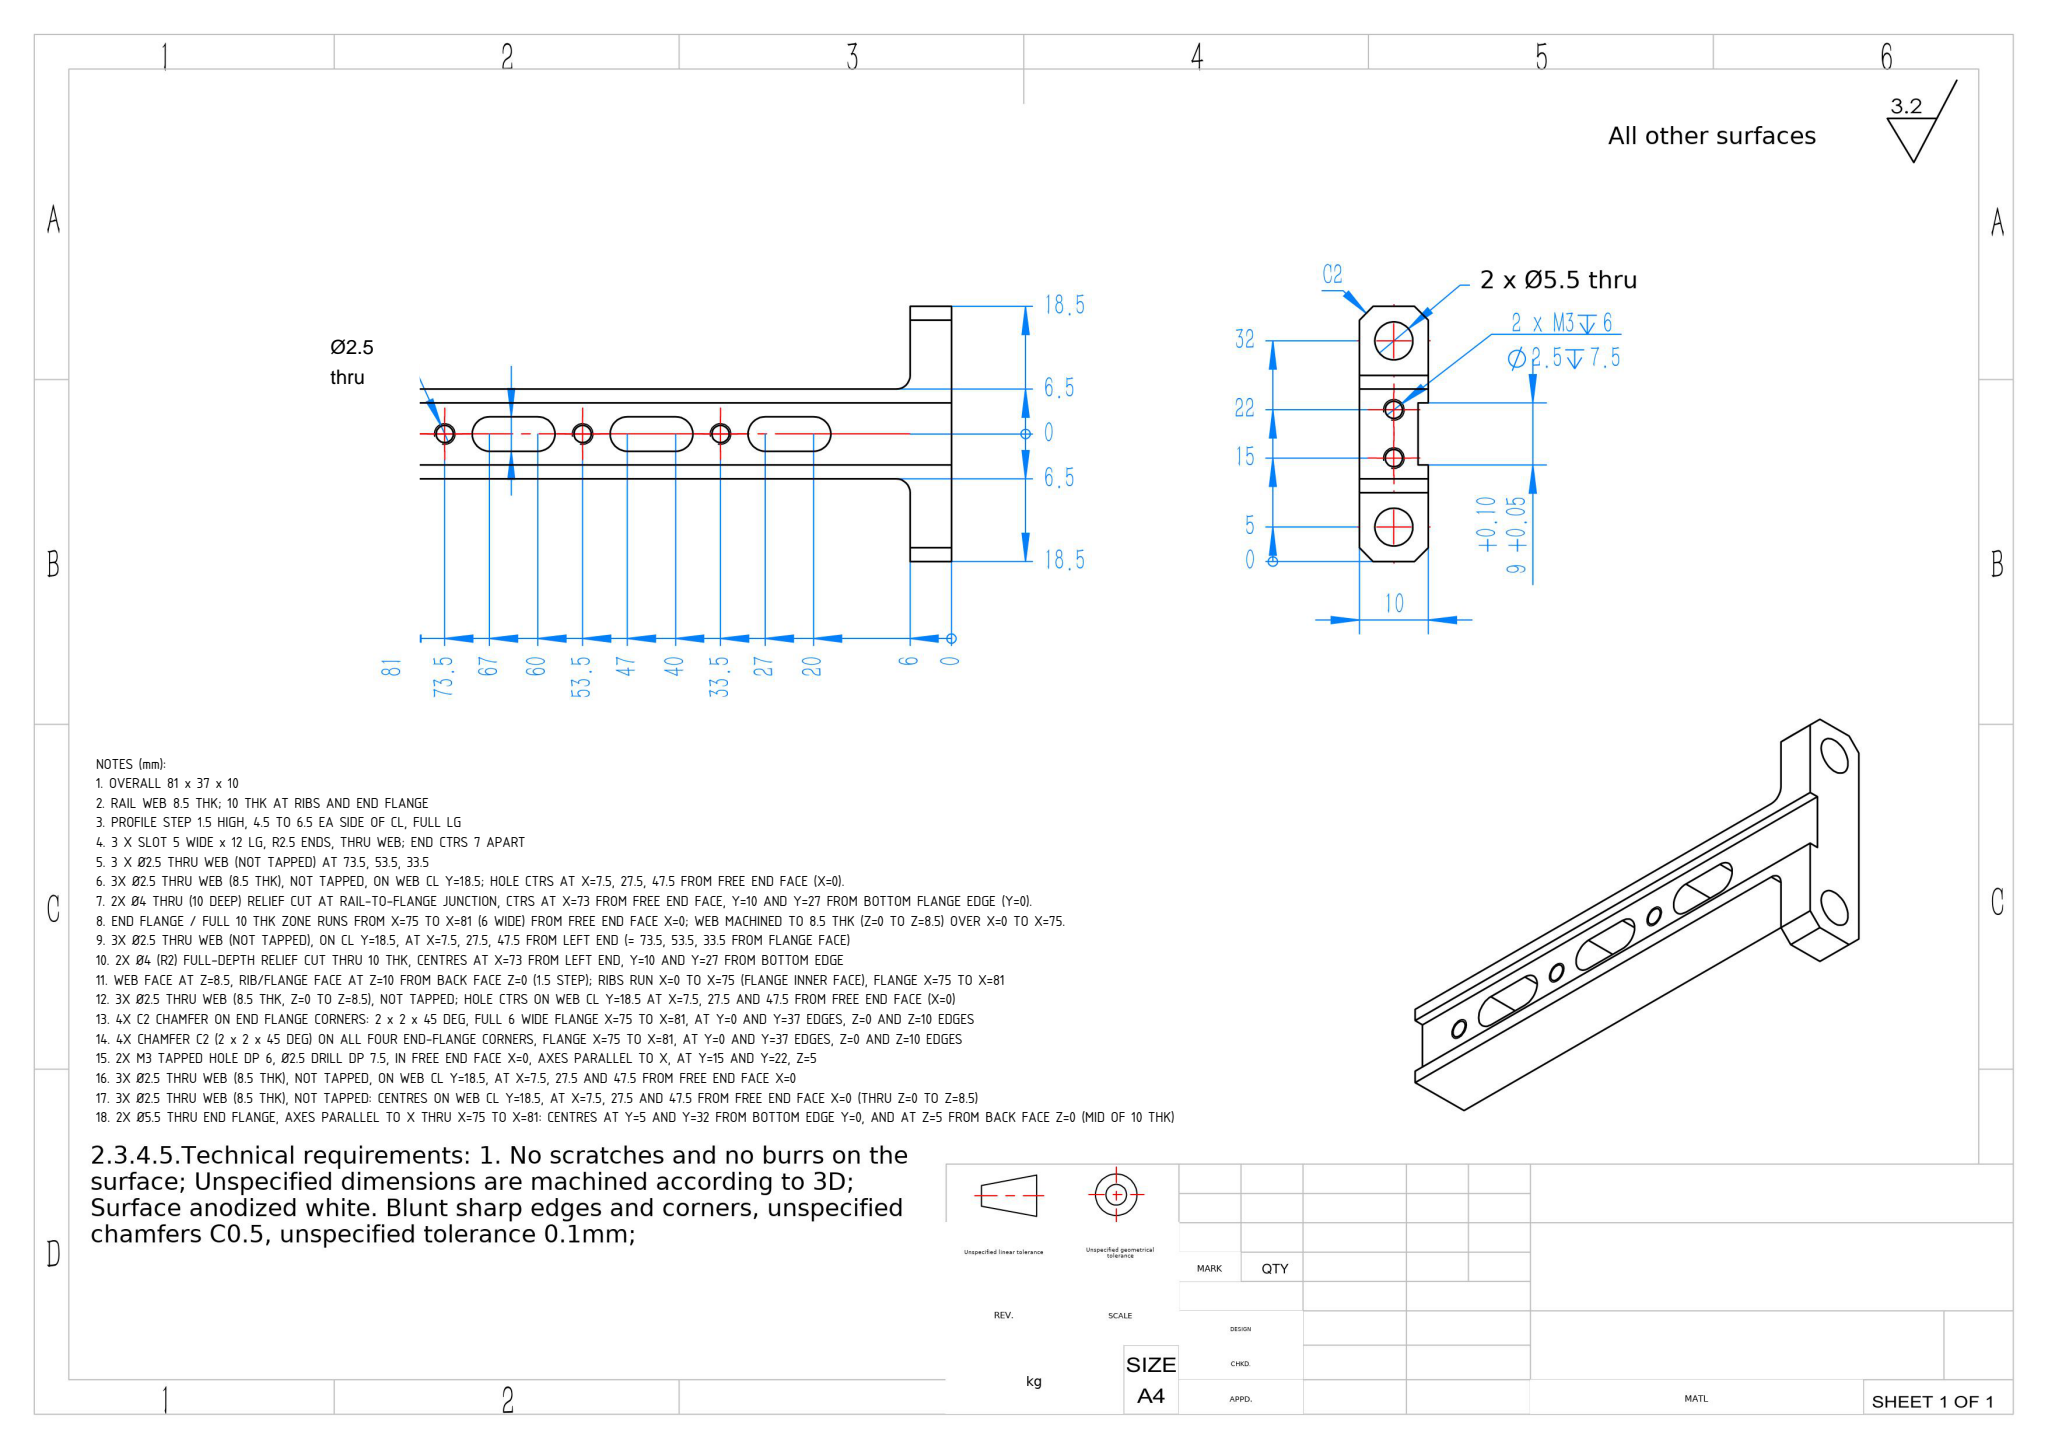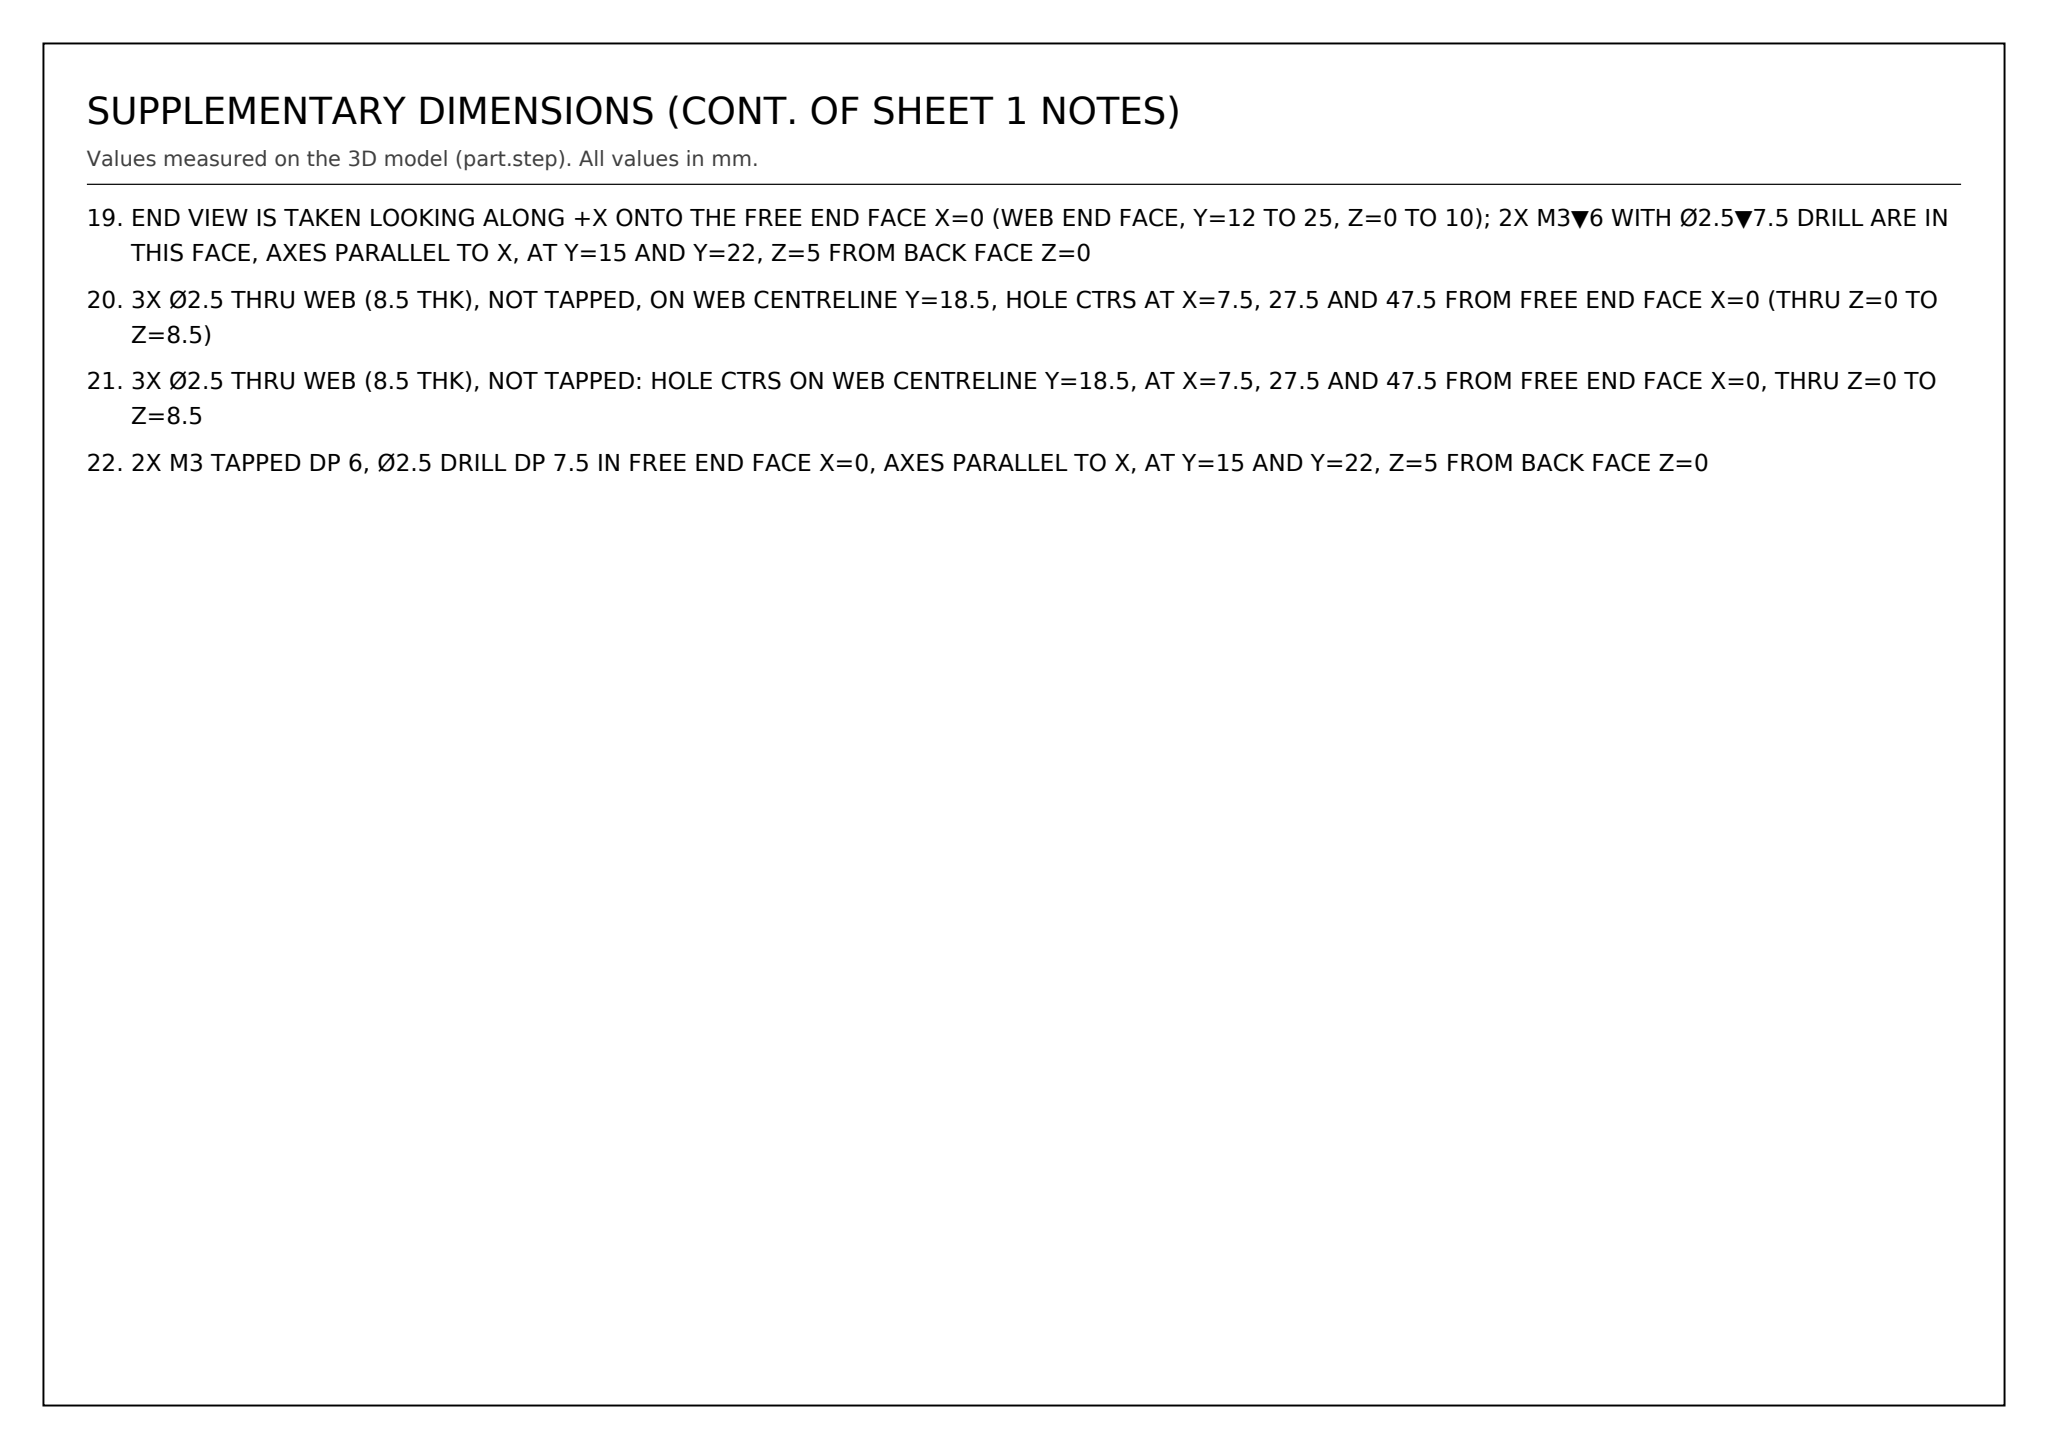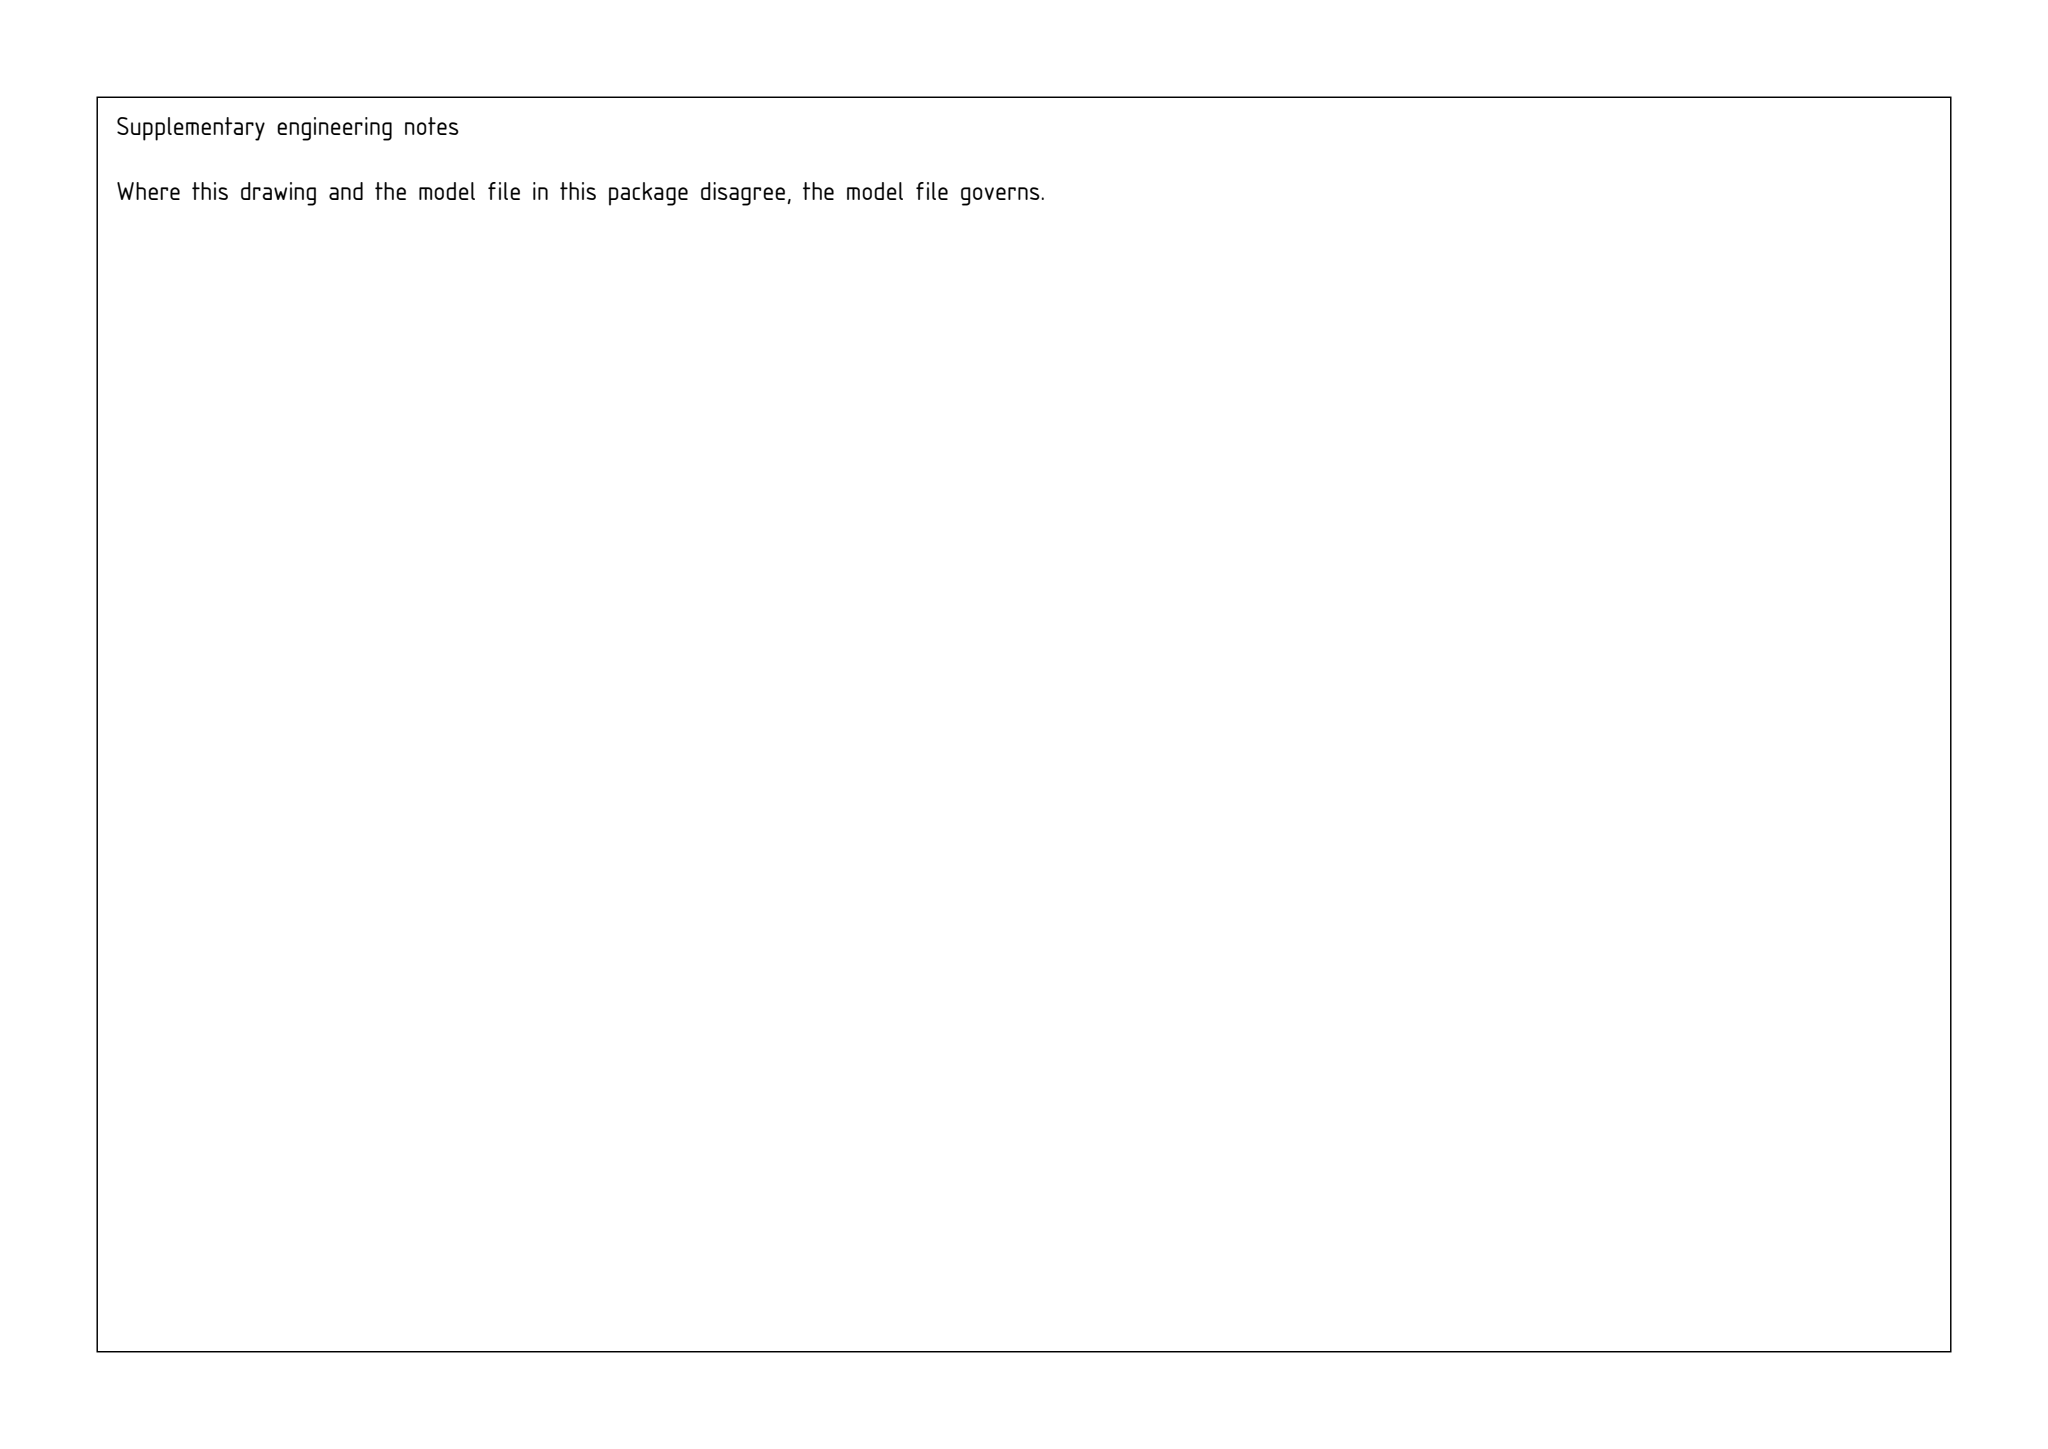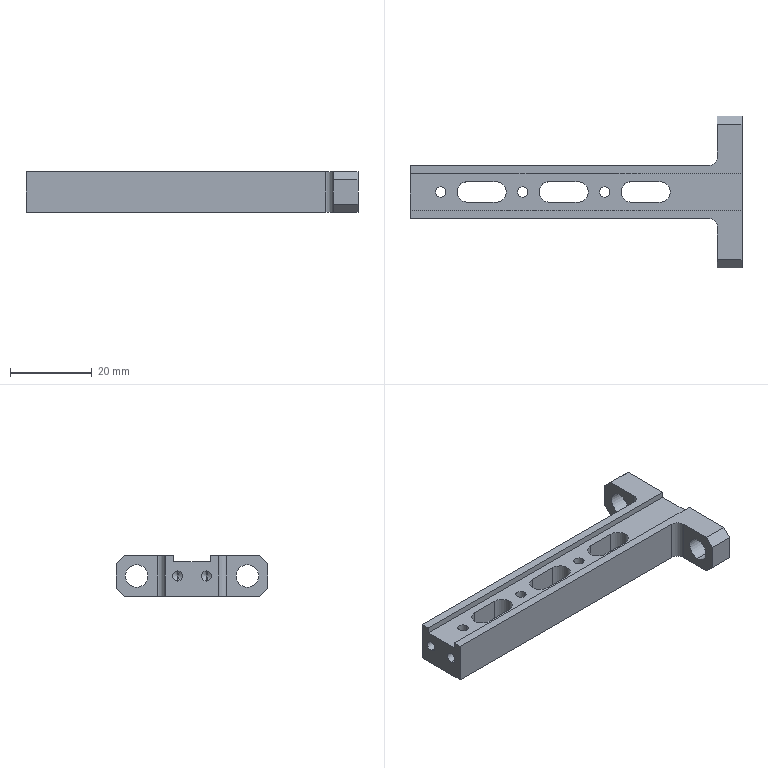Part | SolidWorks | mm | 1 solid | 53 faces | box 81 x 37 x 10 mm | volume 8966 mm3 | cylinder 25 | plane 24 | cone 4 | commonest cylinder face diameters 2.5 x10 5 x9 5.5 x4 4 x2
Drawing notes:
OVERALL 81 x 37 x 10 | from the solid: bbox_xyz 81 x 37 x 10
RAIL WEB 8.5 THK; 10 THK AT RIBS AND END FLANGE | from the solid: z planes 0, 8.5, 10; all z-axis holes/slots 8.5 deep; bbox z=10
PROFILE STEP 1.5 HIGH, 4.5 TO 6.5 EA SIDE OF CL, FULL LG | from the solid: y planes 12/14 and 23/25 (4.5 & 6.5 from CL y=18.5); z 8.5 to 10 = 1.5
3 X SLOT 5 WIDE x 12 LG, R2.5 ENDS, THRU WEB; END CTRS 7 APART | from the solid: Ø5 z-cyls paired x=14/21, 34/41, 54/61, y=18.5, len 8.5; slot walls y=16 & 21
3 X Ø2.5 THRU WEB (NOT TAPPED) AT 73.5, 53.5, 33.5 | from the solid: Ø2.5 z-cyls at x=7.5, 27.5, 47.5, y=18.5, len 8.5 thru; no thread/cbore
3X Ø2.5 THRU WEB (8.5 THK), NOT TAPPED, ON WEB CL Y=18.5; HOLE CTRS AT X=7.5, 27.5, 47.5 FROM FREE END FACE (X=0). | from the solid: cylinders [2.5, z, (7.5,18.5), 8.5], [2.5, z, (27.5,18.5), 8.5], [2.5, z, (47.5,18.5), 8.5]
2X Ø4 THRU (10 DEEP) RELIEF CUT AT RAIL-TO-FLANGE JUNCTION, CTRS AT X=73 FROM FREE END FACE, Y=10 AND Y=27 FROM BOTTOM FLANGE EDGE (Y=0). | from the solid: cylinders [4.0, z, (73.0,10.0), 10.0] and [4.0, z, (73.0,27.0), 10.0]
END FLANGE / FULL 10 THK ZONE RUNS FROM X=75 TO X=81 (6 WIDE) FROM FREE END FACE X=0; WEB MACHINED TO 8.5 THK (Z=0 TO Z=8.5) OVER X=0 TO X=75. | from the solid: axis_planes x=75.0, x=81.0, x=0.0 and z=8.5, z=10.0
3X Ø2.5 THRU WEB (NOT TAPPED), ON CL Y=18.5, AT X=7.5, 27.5, 47.5 FROM LEFT END (= 73.5, 53.5, 33.5 FROM FLANGE FACE) | from the solid: cylinders dia 2.5 axis z at [7.5,18.5], [27.5,18.5], [47.5,18.5], length 8.5 (web thk)
2X Ø4 (R2) FULL-DEPTH RELIEF CUT THRU 10 THK, CENTRES AT X=73 FROM LEFT END, Y=10 AND Y=27 FROM BOTTOM EDGE | from the solid: cylinders dia 4.0 axis z at [73.0,10.0] and [73.0,27.0], length 10.0
WEB FACE AT Z=8.5, RIB/FLANGE FACE AT Z=10 FROM BACK FACE Z=0 (1.5 STEP); RIBS RUN X=0 TO X=75 (FLANGE INNER FACE), FLANGE X=75 TO X=81 | from the solid: axis planes z=8.5 (1), z=10.0 (2), x=0.0, x=75.0 (2), x=81.0
3X Ø2.5 THRU WEB (8.5 THK, Z=0 TO Z=8.5), NOT TAPPED; HOLE CTRS ON WEB CL Y=18.5 AT X=7.5, 27.5 AND 47.5 FROM FREE END FACE (X=0) | from the solid: cylinders dia 2.5 axis z at [7.5,18.5], [27.5,18.5], [47.5,18.5], length 8.5
4X C2 CHAMFER ON END FLANGE CORNERS: 2 x 2 x 45 DEG, FULL 6 WIDE FLANGE X=75 TO X=81, AT Y=0 AND Y=37 EDGES, Z=0 AND Z=10 EDGES | from the solid: inclined_planes: four 45 deg faces, size 6 x 2 x 2, bbox_from [75,0,0], [75,0,8], [75,35,0], [75,35,8]
4X CHAMFER C2 (2 x 2 x 45 DEG) ON ALL FOUR END-FLANGE CORNERS, FLANGE X=75 TO X=81, AT Y=0 AND Y=37 EDGES, Z=0 AND Z=10 EDGES | from the solid: inclined_planes: four 45 deg faces, size 6.0 x 2.0 x 2.0, bbox_from [75,0,0], [75,0,8], [75,35,0], [75,35,8]
2X M3 TAPPED HOLE DP 6, Ø2.5 DRILL DP 7.5, IN FREE END FACE X=0, AXES PARALLEL TO X, AT Y=15 AND Y=22, Z=5 | from the solid: cylinders: hole/bore dia 2.5 axis x at (y=15,z=5) and (y=22,z=5), from x=0 to x=7.5; cones 118 deg ref_dia 2.5 at x=7.5 (drill points)
3X Ø2.5 THRU WEB (8.5 THK), NOT TAPPED, ON WEB CL Y=18.5, AT X=7.5, 27.5 AND 47.5 FROM FREE END FACE X=0 | from the solid: cylinders: hole/bore dia 2.5 axis z at (7.5,18.5), (27.5,18.5), (47.5,18.5), from z=0 to z=8.5
3X Ø2.5 THRU WEB (8.5 THK), NOT TAPPED: CENTRES ON WEB CL Y=18.5, AT X=7.5, 27.5 AND 47.5 FROM FREE END FACE X=0 (THRU Z=0 TO Z=8.5) | from the solid: cylinders: hole/bore Ø2.5 axis z at (7.5,18.5), (27.5,18.5), (47.5,18.5), from z=0 to z=8.5, 360 deg
2X Ø5.5 THRU END FLANGE, AXES PARALLEL TO X THRU X=75 TO X=81: CENTRES AT Y=5 AND Y=32 FROM BOTTOM EDGE Y=0, AND AT Z=5 FROM BACK FACE Z=0 (MID OF 10 THK) | from the solid: cylinders: hole/bore Ø5.5 axis x at [y=32, z=5] and [y=5, z=5], from x=75 to x=81
END VIEW IS TAKEN LOOKING ALONG +X ONTO THE FREE END FACE X=0 (WEB END FACE, Y=12 TO 25, Z=0 TO 10); 2X M3▼6 WITH Ø2.5▼7.5 DRILL ARE IN THIS FACE, AXES PARALLEL TO X, AT Y=15 AND Y=22, Z=5 FROM BACK FACE Z=0 | from the solid: axis_planes: x=0 face extent y[12,25] z[0,10]; cylinders: hole/bore Ø2.5 axis x at [y=15,z=5] and [y=22,z=5], from x=0 to x=7.5
3X Ø2.5 THRU WEB (8.5 THK), NOT TAPPED, ON WEB CENTRELINE Y=18.5, HOLE CTRS AT X=7.5, 27.5 AND 47.5 FROM FREE END FACE X=0 (THRU Z=0 TO Z=8.5) | from the solid: cylinders: hole/bore dia 2.5 axis z at (7.5,18.5), (27.5,18.5), (47.5,18.5), from z=0 to z=8.5, 360 deg
3X Ø2.5 THRU WEB (8.5 THK), NOT TAPPED: HOLE CTRS ON WEB CENTRELINE Y=18.5, AT X=7.5, 27.5 AND 47.5 FROM FREE END FACE X=0, THRU Z=0 TO Z=8.5 | from the solid: cylinders: hole/bore Ø2.5 axis z at (7.5,18.5), (27.5,18.5), (47.5,18.5), from Z=0 to Z=8.5
2X M3 TAPPED DP 6, Ø2.5 DRILL DP 7.5 IN FREE END FACE X=0, AXES PARALLEL TO X, AT Y=15 AND Y=22, Z=5 FROM BACK FACE Z=0 | from the solid: cylinders: hole/bore Ø2.5 axis x at (y=15,z=5) and (y=22,z=5), from X=0 to X=7.5; cones 118° ref dia 2.5 at x=7.5
build123d program:
from build123d import *

# Parameters (mm, degrees)
SKETCH1_W                  = 75
SKETCH1_H                  = 13
BOSS_EXTRUDE1_DEPTH        = 10
SKETCH2_W                  = 75
SKETCH2_H                  = 9
CUT_EXTRUDE1_DEPTH         = 1.5
SKETCH6_W                  = 10
SKETCH6_H                  = 37
BOSS_EXTRUDE2_DEPTH        = 6
M3_TAPPED_HOLE1_D          = 2.5
F_5_5_5_5_DIAMETER_HOLE1_D = 5.5
CHAMFER1_SIZE              = 2
SKETCH14_W                 = 11
SKETCH14_H                 = 9
CUT_EXTRUDE2_DEPTH         = 10
M3_TAPPED_HOLE2_D          = 2.5
M3_TAPPED_HOLE2_DEPTH      = 7.5
M3_TAPPED_HOLE2_TIP        = 0.7511
FILLET1_R                  = 2
CUT_EXTRUDE3_DEPTH         = 49.317
LPATTERN1_COUNT            = 3
LPATTERN1_PITCH            = 20


with BuildPart() as part:
    # Sketch1 → Boss-Extrude1 (new body)
    with BuildSketch(Plane.XY):
        Rectangle(SKETCH1_W, SKETCH1_H)
    extrude(amount=BOSS_EXTRUDE1_DEPTH)

    # Sketch2 → Cut-Extrude1 (cut)
    with BuildSketch(Plane.XY.offset(10)):
        Rectangle(SKETCH2_W, SKETCH2_H)
    extrude(amount=-CUT_EXTRUDE1_DEPTH, mode=Mode.SUBTRACT)

    # Sketch6 → Boss-Extrude2 (add)
    with BuildSketch(Plane(origin=(37.5, 0, 0), x_dir=(0, 0, -1), z_dir=(1, 0, 0))):
        with Locations((-5, 0)):
            Rectangle(SKETCH6_W, SKETCH6_H)
    extrude(amount=BOSS_EXTRUDE2_DEPTH)

    # M3 Tapped Hole1 (through all)
    with Locations(Plane.XY.offset(8.5)):
        with Locations((10, 0), (-10, 0), (-30, 0)):
            Hole(M3_TAPPED_HOLE1_D / 2)

    # 5.5 _5.5_ Diameter Hole1 (through all)
    with Locations(Plane.ZY.offset(-37.5)):
        with Locations((5, 13.5), (5, -13.5)):
            Hole(F_5_5_5_5_DIAMETER_HOLE1_D / 2)

    # Chamfer1
    chamfer1_edges = [part.edges().sort_by_distance(p)[0] for p in [
        (40.5, -18.5, 0),
        (40.5, 18.5, 0),
        (40.5, 18.5, 10),
        (40.5, -18.5, 10),
    ]]
    chamfer(chamfer1_edges, length=CHAMFER1_SIZE)

    # Sketch14 → Cut-Extrude2 (cut)
    with BuildSketch(Plane.XY.offset(8.5)):
        with Locations((38, 0)):
            Rectangle(SKETCH14_W, SKETCH14_H)
    extrude(amount=CUT_EXTRUDE2_DEPTH, mode=Mode.SUBTRACT)

    # M3 Tapped Hole2
    with Locations(Plane.ZY.offset(37.5)):
        with Locations((5, -3.5), (5, 3.5)):
            Hole(M3_TAPPED_HOLE2_D / 2, depth=M3_TAPPED_HOLE2_DEPTH)
            with Locations((0, 0, -(M3_TAPPED_HOLE2_DEPTH + M3_TAPPED_HOLE2_TIP / 2))):  # 118° drill point
                Cone(0, M3_TAPPED_HOLE2_D / 2, M3_TAPPED_HOLE2_TIP, mode=Mode.SUBTRACT)

    # Fillet1
    fillet1_edges = [part.edges().sort_by_distance(p)[0] for p in [
        (37.5, -6.5, 5),
        (37.5, 6.5, 5),
    ]]
    fillet(fillet1_edges, radius=FILLET1_R)

    # Sketch18 → Cut-Extrude3 (cut, through all)
    with BuildSketch(Plane(origin=(0, 0, 0), x_dir=(-1, 0, 0), z_dir=(0, 0, -1))):
        with BuildLine():
            Line((16.5, 2.5), (23.5, 2.5))
            ThreePointArc((23.5, 2.5), (26, 0), (23.5, -2.5))
            Line((23.5, -2.5), (16.5, -2.5))
            ThreePointArc((16.5, -2.5), (14, 0), (16.5, 2.5))
        make_face()
    cut_extrude3 = extrude(amount=-CUT_EXTRUDE3_DEPTH, mode=Mode.SUBTRACT)

    # LPattern1: Cut-Extrude3 ×3
    with Locations(*[(i * LPATTERN1_PITCH, 0, 0) for i in range(1, LPATTERN1_COUNT)]):
        add(cut_extrude3, mode=Mode.SUBTRACT)


solid = part.part